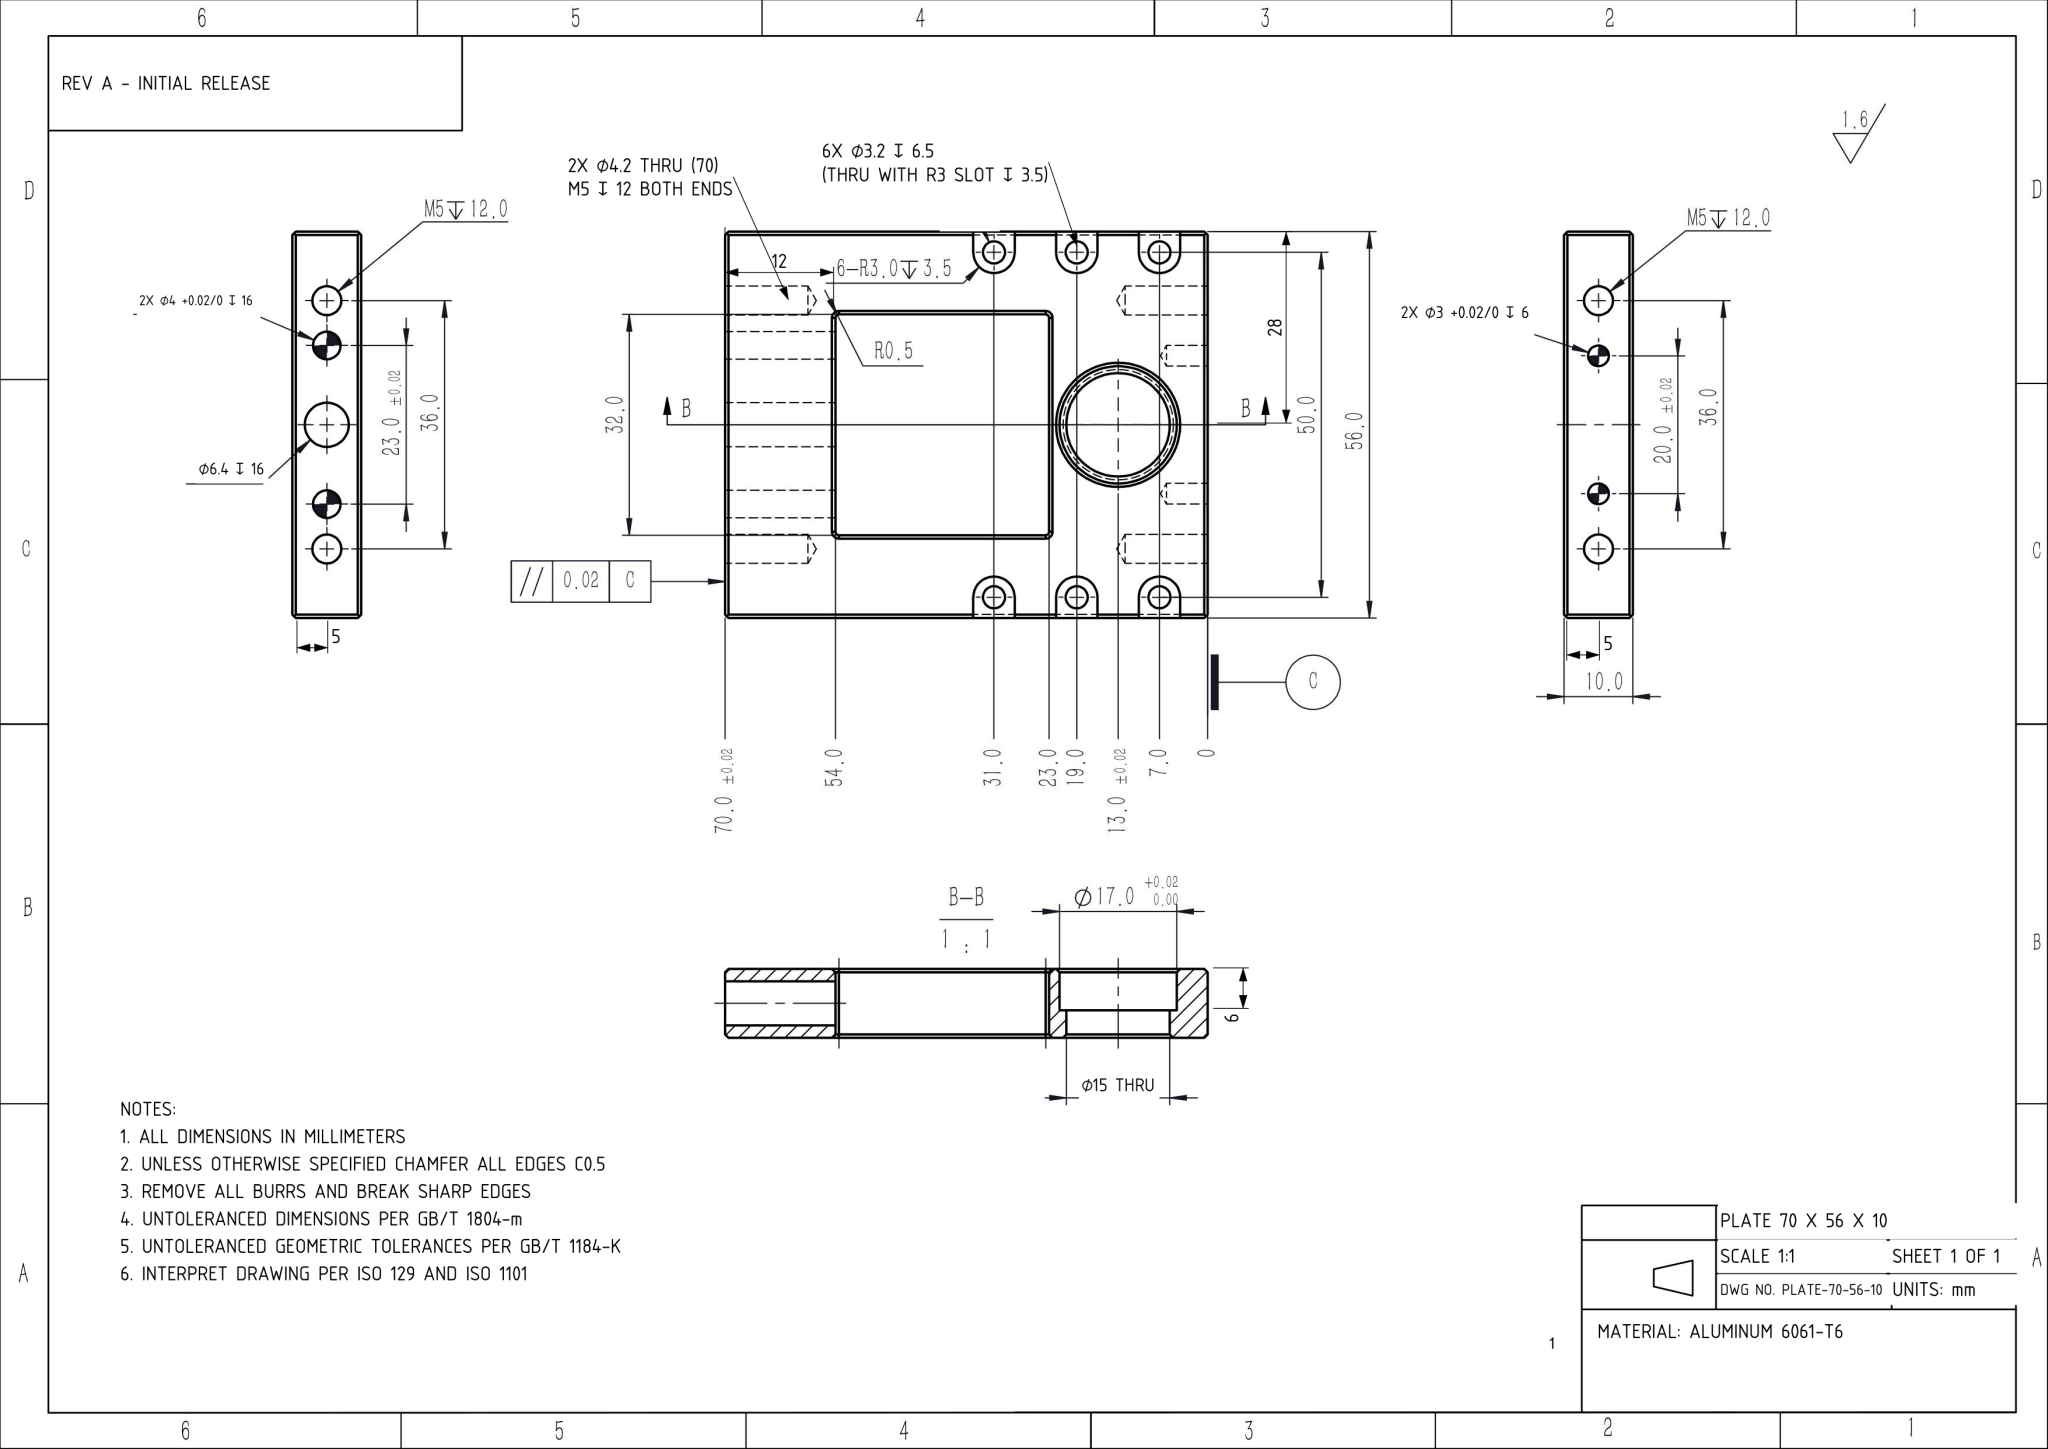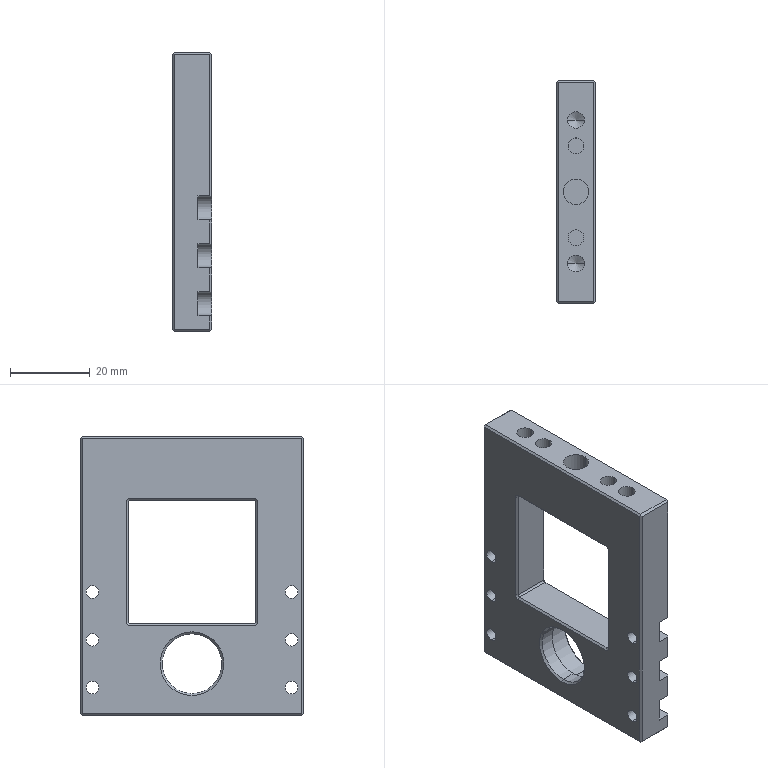Part | NX | mm | 1 solid | 123 faces | box 10 x 56 x 70 mm | volume 24425 mm3 | plane 55 | cylinder 44 | cone 24 | commonest cylinder face diameters 3.2 x12 4.2 x8 6 x6 3 x4 4 x4 1 x4 6.4 x2 15 x2